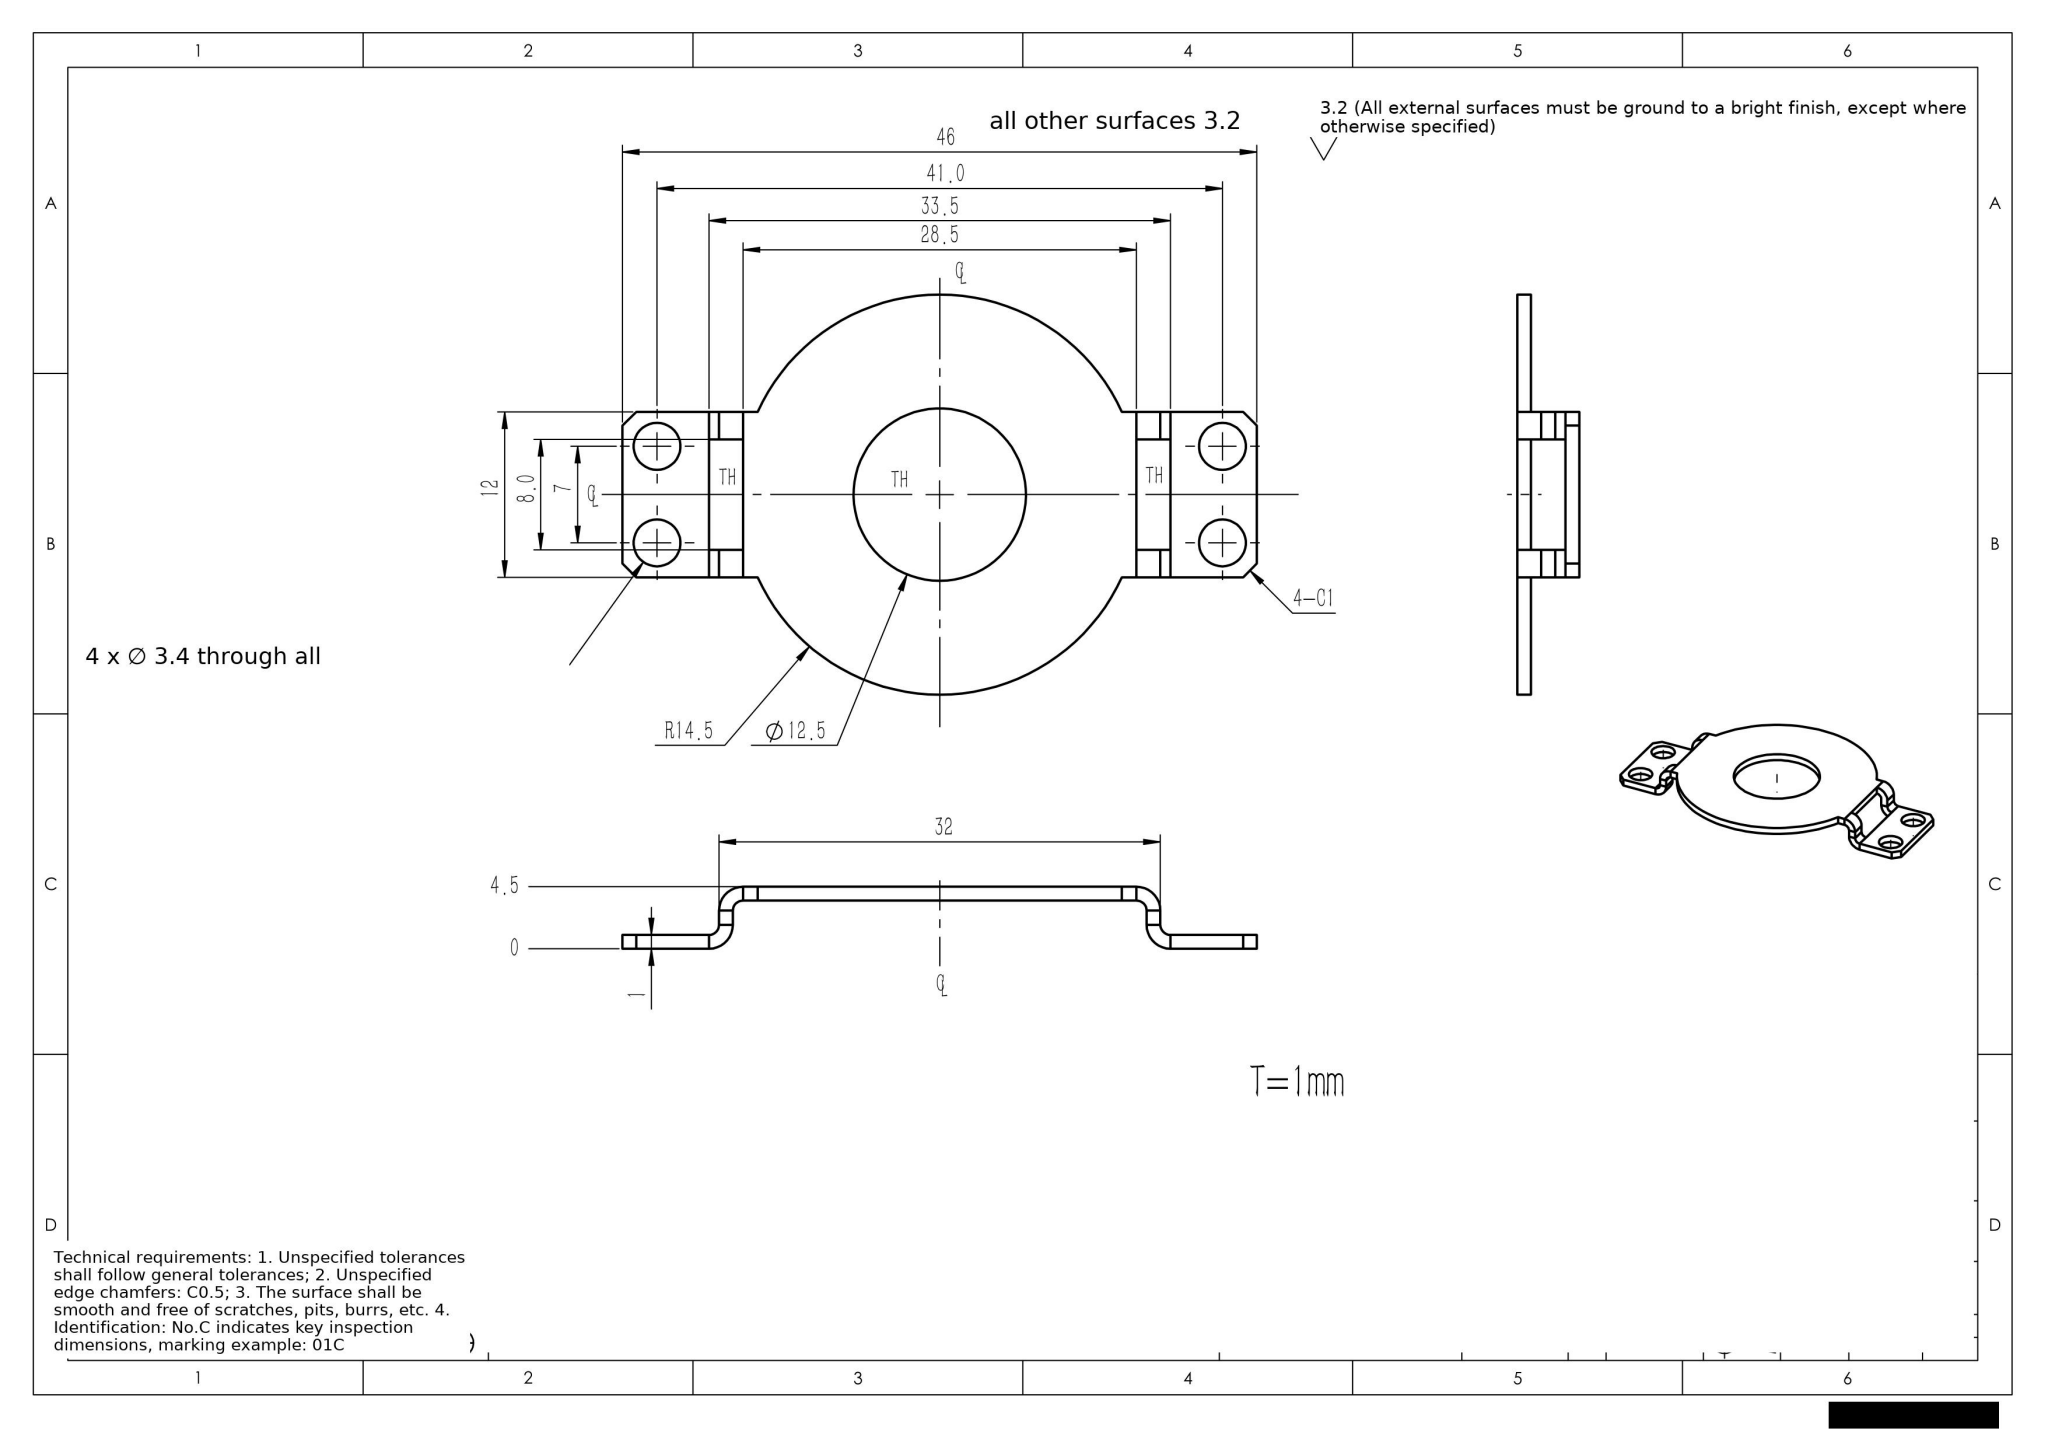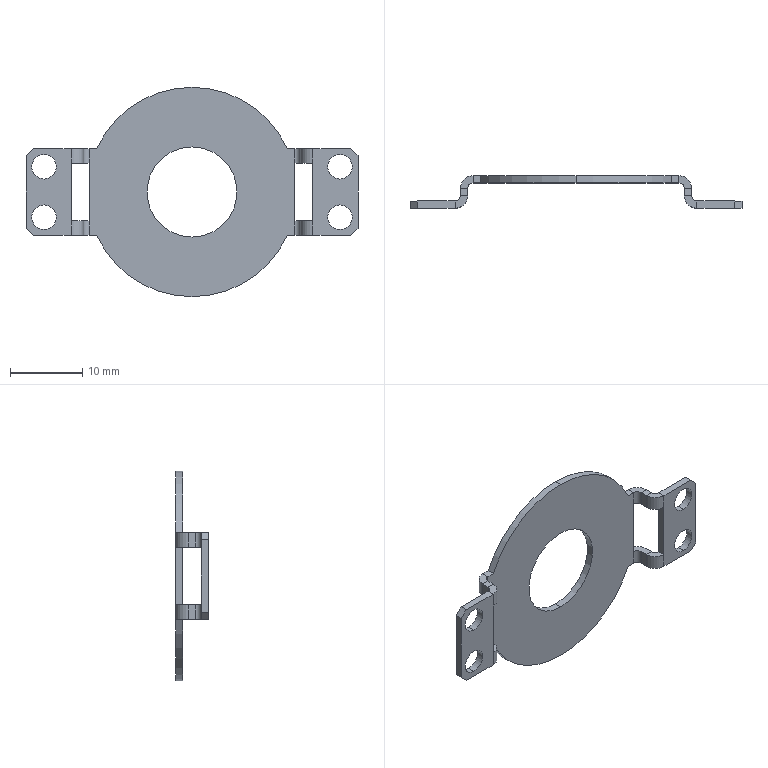Part | SolidWorks | mm | 1 solid | 79 faces | box 46 x 4.5 x 29 mm | volume 694 mm3 | plane 50 | cylinder 29 | commonest cylinder face diameters 3.4 x8 3.473 x8 1.473 x8 29 x3 12.5 x2